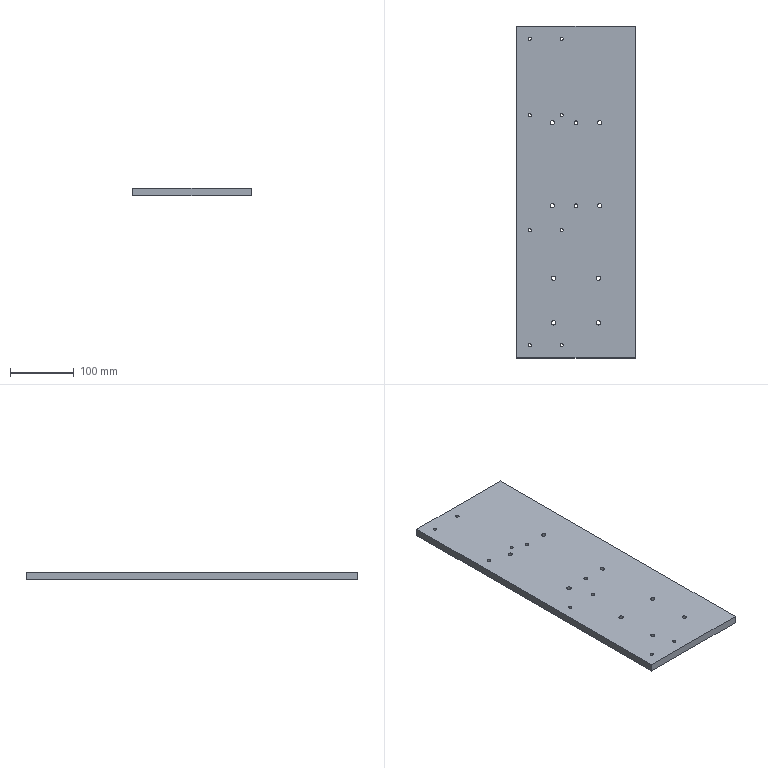Component | SolidWorks | Y-AxisSlideMountingPlate-1 | 1 solid | 42 faces | box 185 x 520 x 12 mm | volume 1148350 mm3 | cylinder 36 | plane 6 | commonest cylinder face diameters 6.8 x16 5 x16 6 x4